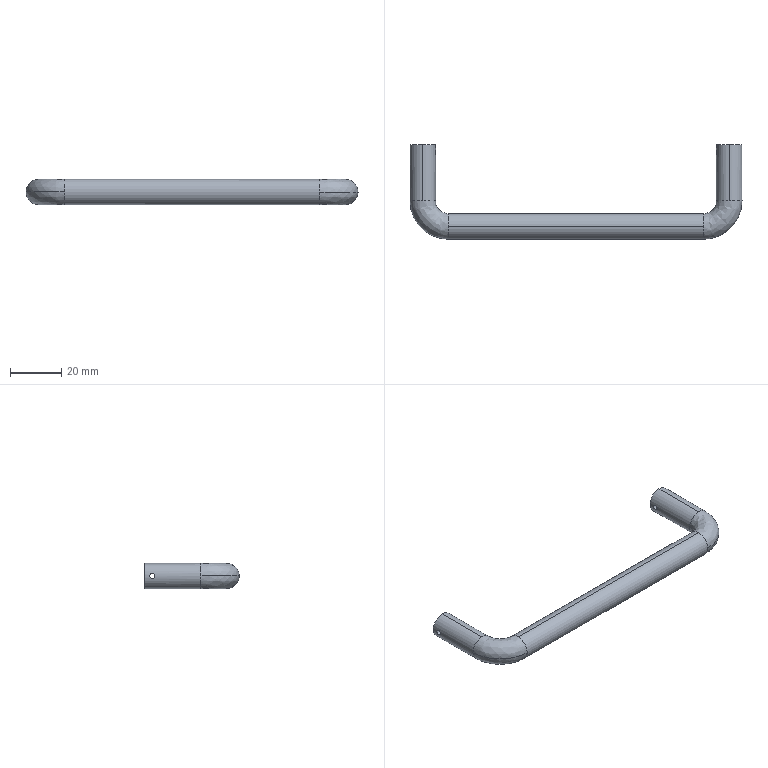Component | SolidWorks | ControlAssembly-1_UWAFN120-1_2_1-1 | 1 solid | 16 faces | box 130 x 37 x 10.01 mm | volume 13715 mm3 | cylinder 10 | spline 4 | plane 2 | commonest cylinder face diameters 10 x6 2 x4
STEP:
#1=COLOUR_RGB('',0.7922,0.8196,0.9333);
#2=FILL_AREA_STYLE_COLOUR('',#1);
#3=FILL_AREA_STYLE('',(#2));
#4=SURFACE_STYLE_FILL_AREA(#3);
#5=SURFACE_SIDE_STYLE('',(#4));
#6=SURFACE_STYLE_USAGE(.BOTH.,#5);
#7=PRESENTATION_STYLE_ASSIGNMENT((#6));
#8=CARTESIAN_POINT('',(19.707,0.8097,21.042));
#9=VERTEX_POINT('',#8);
#10=CARTESIAN_POINT('',(19.707,0.8097,21.121));
#11=VERTEX_POINT('',#10);
#12=CARTESIAN_POINT('',(19.707,0.8097,21.042));
#13=CARTESIAN_POINT('',(19.707,0.8149,21.042));
#14=CARTESIAN_POINT('',(19.707,0.82,21.043));
#15=CARTESIAN_POINT('',(19.706,0.8295,21.047));
#16=CARTESIAN_POINT('',(19.706,0.8339,21.05));
#17=CARTESIAN_POINT('',(19.705,0.8412,21.057));
#18=CARTESIAN_POINT('',(19.704,0.8441,21.061));
#19=CARTESIAN_POINT('',(19.703,0.848,21.071));
#20=CARTESIAN_POINT('',(19.703,0.8491,21.076));
#21=CARTESIAN_POINT('',(19.703,0.8491,21.086));
#22=CARTESIAN_POINT('',(19.703,0.848,21.092));
#23=CARTESIAN_POINT('',(19.704,0.8441,21.101));
#24=CARTESIAN_POINT('',(19.705,0.8411,21.105));
#25=CARTESIAN_POINT('',(19.706,0.8339,21.113));
#26=CARTESIAN_POINT('',(19.706,0.8295,21.116));
#27=CARTESIAN_POINT('',(19.707,0.82,21.12));
#28=CARTESIAN_POINT('',(19.707,0.8149,21.121));
#29=CARTESIAN_POINT('',(19.707,0.8097,21.121));
#30=B_SPLINE_CURVE_WITH_KNOTS('',3,(#12,#13,#14,#15,#16,#17,#18,#19,#20,#21,#22,#23,#24,#25,#26,#27,#28,#29),.UNSPECIFIED.,.F.,.F.,(4,2,2,2,2,2,2,2,4),(0.004702,0.005093,0.005485,0.005877,0.006269,0.00666,0.007052,0.007444,0.007836),.UNSPECIFIED.);
#31=EDGE_CURVE('',#9,#11,#30,.T.);
#32=ORIENTED_EDGE('',*,*,#31,.F.);
#33=CARTESIAN_POINT('',(20.093,0.8097,21.042));
#34=VERTEX_POINT('',#33);
#35=CARTESIAN_POINT('',(19.703,0.8097,21.042));
#36=DIRECTION('',(1.,0.,-0.00009864));
#37=VECTOR('',#36,39.37);
#38=LINE('',#35,#37);
#39=EDGE_CURVE('',#9,#34,#38,.T.);
#40=ORIENTED_EDGE('',*,*,#39,.T.);
#41=CARTESIAN_POINT('',(20.093,0.8097,21.121));
#42=VERTEX_POINT('',#41);
#43=CARTESIAN_POINT('',(20.093,0.8097,21.121));
#44=CARTESIAN_POINT('',(20.093,0.8149,21.121));
#45=CARTESIAN_POINT('',(20.093,0.82,21.119));
#46=CARTESIAN_POINT('',(20.094,0.8296,21.116));
#47=CARTESIAN_POINT('',(20.094,0.8339,21.113));
#48=CARTESIAN_POINT('',(20.095,0.8412,21.105));
#49=CARTESIAN_POINT('',(20.096,0.8441,21.101));
#50=CARTESIAN_POINT('',(20.097,0.848,21.091));
#51=CARTESIAN_POINT('',(20.097,0.8491,21.086));
#52=CARTESIAN_POINT('',(20.097,0.8491,21.076));
#53=CARTESIAN_POINT('',(20.097,0.848,21.071));
#54=CARTESIAN_POINT('',(20.096,0.8441,21.061));
#55=CARTESIAN_POINT('',(20.095,0.8412,21.057));
#56=CARTESIAN_POINT('',(20.094,0.8339,21.05));
#57=CARTESIAN_POINT('',(20.094,0.8295,21.047));
#58=CARTESIAN_POINT('',(20.093,0.82,21.043));
#59=CARTESIAN_POINT('',(20.093,0.8148,21.042));
#60=CARTESIAN_POINT('',(20.093,0.8097,21.042));
#61=B_SPLINE_CURVE_WITH_KNOTS('',3,(#43,#44,#45,#46,#47,#48,#49,#50,#51,#52,#53,#54,#55,#56,#57,#58,#59,#60),.UNSPECIFIED.,.F.,.F.,(4,2,2,2,2,2,2,2,4),(0.,0.0003918,0.0007836,0.001175,0.001567,0.001959,0.002351,0.002743,0.003134),.UNSPECIFIED.);
#62=EDGE_CURVE('',#42,#34,#61,.T.);
#63=ORIENTED_EDGE('',*,*,#62,.F.);
#64=CARTESIAN_POINT('',(19.703,0.8097,21.121));
#65=DIRECTION('',(1.,0.,-0.00009864));
#66=VECTOR('',#65,39.37);
#67=LINE('',#64,#66);
#68=EDGE_CURVE('',#11,#42,#67,.T.);
#69=ORIENTED_EDGE('',*,*,#68,.F.);
#70=EDGE_LOOP('',(#32,#40,#63,#69));
#71=FACE_OUTER_BOUND('',#70,.T.);
#72=CARTESIAN_POINT('',(19.703,0.8097,21.081));
#73=DIRECTION('',(1.,0.,-0.00009864));
#74=DIRECTION('',(0.00009864,0.,1.));
#75=AXIS2_PLACEMENT_3D('',#72,#73,#74);
#76=CYLINDRICAL_SURFACE('',#75,0.03937);
#77=ADVANCED_FACE('',(#71),#76,.F.);
#78=CARTESIAN_POINT('',(24.431,0.8097,21.041));
#79=VERTEX_POINT('',#78);
#80=CARTESIAN_POINT('',(24.431,0.8097,21.12));
#81=VERTEX_POINT('',#80);
#82=CARTESIAN_POINT('',(24.431,0.8097,21.041));
#83=CARTESIAN_POINT('',(24.431,0.8148,21.041));
#84=CARTESIAN_POINT('',(24.431,0.82,21.042));
#85=CARTESIAN_POINT('',(24.43,0.8295,21.046));
#86=CARTESIAN_POINT('',(24.43,0.8339,21.049));
#87=CARTESIAN_POINT('',(24.429,0.8412,21.056));
#88=CARTESIAN_POINT('',(24.428,0.8441,21.061));
#89=CARTESIAN_POINT('',(24.428,0.848,21.07));
#90=CARTESIAN_POINT('',(24.427,0.8491,21.075));
#91=CARTESIAN_POINT('',(24.427,0.8491,21.086));
#92=CARTESIAN_POINT('',(24.428,0.848,21.091));
#93=CARTESIAN_POINT('',(24.428,0.8441,21.101));
#94=CARTESIAN_POINT('',(24.429,0.8412,21.105));
#95=CARTESIAN_POINT('',(24.43,0.8339,21.112));
#96=CARTESIAN_POINT('',(24.43,0.8296,21.115));
#97=CARTESIAN_POINT('',(24.431,0.8201,21.119));
#98=CARTESIAN_POINT('',(24.431,0.8149,21.12));
#99=CARTESIAN_POINT('',(24.431,0.8097,21.12));
#100=B_SPLINE_CURVE_WITH_KNOTS('',3,(#82,#83,#84,#85,#86,#87,#88,#89,#90,#91,#92,#93,#94,#95,#96,#97,#98,#99),.UNSPECIFIED.,.F.,.F.,(4,2,2,2,2,2,2,2,4),(0.003134,0.003526,0.003918,0.004309,0.004701,0.005093,0.005485,0.005876,0.006268),.UNSPECIFIED.);
#101=EDGE_CURVE('',#79,#81,#100,.T.);
#102=ORIENTED_EDGE('',*,*,#101,.F.);
#103=CARTESIAN_POINT('',(24.817,0.8097,21.041));
#104=VERTEX_POINT('',#103);
#105=CARTESIAN_POINT('',(19.703,0.8097,21.042));
#106=DIRECTION('',(1.,0.,-0.00009864));
#107=VECTOR('',#106,39.37);
#108=LINE('',#105,#107);
#109=EDGE_CURVE('',#79,#104,#108,.T.);
#110=ORIENTED_EDGE('',*,*,#109,.T.);
#111=CARTESIAN_POINT('',(24.817,0.8097,21.12));
#112=VERTEX_POINT('',#111);
#113=CARTESIAN_POINT('',(24.817,0.8097,21.12));
#114=CARTESIAN_POINT('',(24.817,0.8149,21.12));
#115=CARTESIAN_POINT('',(24.817,0.82,21.119));
#116=CARTESIAN_POINT('',(24.818,0.8296,21.115));
#117=CARTESIAN_POINT('',(24.819,0.8339,21.112));
#118=CARTESIAN_POINT('',(24.82,0.8412,21.105));
#119=CARTESIAN_POINT('',(24.82,0.8441,21.101));
#120=CARTESIAN_POINT('',(24.821,0.848,21.091));
#121=CARTESIAN_POINT('',(24.821,0.8491,21.086));
#122=CARTESIAN_POINT('',(24.821,0.8491,21.076));
#123=CARTESIAN_POINT('',(24.821,0.848,21.07));
#124=CARTESIAN_POINT('',(24.82,0.8441,21.061));
#125=CARTESIAN_POINT('',(24.82,0.8412,21.056));
#126=CARTESIAN_POINT('',(24.819,0.8339,21.049));
#127=CARTESIAN_POINT('',(24.818,0.8295,21.046));
#128=CARTESIAN_POINT('',(24.817,0.82,21.042));
#129=CARTESIAN_POINT('',(24.817,0.8148,21.041));
#130=CARTESIAN_POINT('',(24.817,0.8097,21.041));
#131=B_SPLINE_CURVE_WITH_KNOTS('',3,(#113,#114,#115,#116,#117,#118,#119,#120,#121,#122,#123,#124,#125,#126,#127,#128,#129,#130),.UNSPECIFIED.,.F.,.F.,(4,2,2,2,2,2,2,2,4),(0.,0.0003918,0.0007836,0.001175,0.001567,0.001959,0.002351,0.002743,0.003134),.UNSPECIFIED.);
#132=EDGE_CURVE('',#112,#104,#131,.T.);
#133=ORIENTED_EDGE('',*,*,#132,.F.);
#134=CARTESIAN_POINT('',(19.703,0.8097,21.121));
#135=DIRECTION('',(1.,0.,-0.00009864));
#136=VECTOR('',#135,39.37);
#137=LINE('',#134,#136);
#138=EDGE_CURVE('',#81,#112,#137,.T.);
#139=ORIENTED_EDGE('',*,*,#138,.F.);
#140=EDGE_LOOP('',(#102,#110,#133,#139));
#141=FACE_OUTER_BOUND('',#140,.T.);
#142=CARTESIAN_POINT('',(19.703,0.8097,21.081));
#143=DIRECTION('',(1.,0.,-0.00009864));
#144=DIRECTION('',(0.00009864,0.,1.));
#145=AXIS2_PLACEMENT_3D('',#142,#143,#144);
#146=CYLINDRICAL_SURFACE('',#145,0.03937);
#147=ADVANCED_FACE('',(#141),#146,.F.);
#148=CARTESIAN_POINT('',(24.231,-0.5289,21.081));
#149=VERTEX_POINT('',#148);
#150=CARTESIAN_POINT('',(24.231,-0.332,21.278));
#151=VERTEX_POINT('',#150);
#152=CARTESIAN_POINT('',(24.231,-0.332,21.081));
#153=DIRECTION('',(-1.,-0.,0.00009864));
#154=DIRECTION('',(-0.00009864,-0.,-1.));
#155=AXIS2_PLACEMENT_3D('',#152,#153,#154);
#156=CIRCLE('',#155,0.1969);
#157=EDGE_CURVE('',#149,#151,#156,.T.);
#158=ORIENTED_EDGE('',*,*,#157,.T.);
#159=CARTESIAN_POINT('',(20.294,-0.332,21.278));
#160=VERTEX_POINT('',#159);
#161=CARTESIAN_POINT('',(22.262,-0.332,21.278));
#162=DIRECTION('',(-1.,-0.,0.00009864));
#163=VECTOR('',#162,39.37);
#164=LINE('',#161,#163);
#165=EDGE_CURVE('',#151,#160,#164,.T.);
#166=ORIENTED_EDGE('',*,*,#165,.T.);
#167=CARTESIAN_POINT('',(20.294,-0.5289,21.081));
#168=VERTEX_POINT('',#167);
#169=CARTESIAN_POINT('',(20.294,-0.332,21.081));
#170=DIRECTION('',(1.,0.,-0.00009864));
#171=DIRECTION('',(-0.00009864,-0.,-1.));
#172=AXIS2_PLACEMENT_3D('',#169,#170,#171);
#173=CIRCLE('',#172,0.1969);
#174=EDGE_CURVE('',#160,#168,#173,.T.);
#175=ORIENTED_EDGE('',*,*,#174,.T.);
#176=CARTESIAN_POINT('',(20.294,-0.332,20.884));
#177=VERTEX_POINT('',#176);
#178=CARTESIAN_POINT('',(20.294,-0.332,21.081));
#179=DIRECTION('',(1.,0.,-0.00009864));
#180=DIRECTION('',(-0.00009864,-0.,-1.));
#181=AXIS2_PLACEMENT_3D('',#178,#179,#180);
#182=CIRCLE('',#181,0.1969);
#183=EDGE_CURVE('',#168,#177,#182,.T.);
#184=ORIENTED_EDGE('',*,*,#183,.T.);
#185=CARTESIAN_POINT('',(24.231,-0.332,20.884));
#186=VERTEX_POINT('',#185);
#187=CARTESIAN_POINT('',(22.262,-0.332,20.884));
#188=DIRECTION('',(-1.,-0.,0.00009864));
#189=VECTOR('',#188,39.37);
#190=LINE('',#187,#189);
#191=EDGE_CURVE('',#186,#177,#190,.T.);
#192=ORIENTED_EDGE('',*,*,#191,.F.);
#193=CARTESIAN_POINT('',(24.231,-0.332,21.081));
#194=DIRECTION('',(-1.,-0.,0.00009864));
#195=DIRECTION('',(-0.00009864,-0.,-1.));
#196=AXIS2_PLACEMENT_3D('',#193,#194,#195);
#197=CIRCLE('',#196,0.1969);
#198=EDGE_CURVE('',#186,#149,#197,.T.);
#199=ORIENTED_EDGE('',*,*,#198,.T.);
#200=EDGE_LOOP('',(#158,#166,#175,#184,#192,#199));
#201=FACE_OUTER_BOUND('',#200,.T.);
#202=CARTESIAN_POINT('',(22.262,-0.332,21.081));
#203=DIRECTION('',(-1.,-0.,0.00009864));
#204=DIRECTION('',(-0.00009864,-0.,-1.));
#205=AXIS2_PLACEMENT_3D('',#202,#203,#204);
#206=CYLINDRICAL_SURFACE('',#205,0.1969);
#207=ADVANCED_FACE('',(#201),#206,.T.);
#208=CARTESIAN_POINT('',(24.231,-0.1352,21.081));
#209=VERTEX_POINT('',#208);
#210=CARTESIAN_POINT('',(24.231,-0.332,21.081));
#211=DIRECTION('',(-1.,-0.,0.00009864));
#212=DIRECTION('',(-0.00009864,-0.,-1.));
#213=AXIS2_PLACEMENT_3D('',#210,#211,#212);
#214=CIRCLE('',#213,0.1969);
#215=EDGE_CURVE('',#209,#186,#214,.T.);
#216=ORIENTED_EDGE('',*,*,#215,.F.);
#217=CARTESIAN_POINT('',(24.427,0.06167,21.081));
#218=VERTEX_POINT('',#217);
#219=CARTESIAN_POINT('',(24.231,0.06167,21.081));
#220=DIRECTION('',(0.00009864,0.,1.));
#221=DIRECTION('',(-1.,0.,0.00009864));
#222=AXIS2_PLACEMENT_3D('',#219,#220,#221);
#223=CIRCLE('',#222,0.1969);
#224=EDGE_CURVE('',#209,#218,#223,.T.);
#225=ORIENTED_EDGE('',*,*,#224,.T.);
#226=CARTESIAN_POINT('',(24.624,0.06167,20.884));
#227=VERTEX_POINT('',#226);
#228=CARTESIAN_POINT('',(24.624,0.06167,21.081));
#229=DIRECTION('',(-0.,-1.,0.));
#230=DIRECTION('',(1.,-0.,-0.00009864));
#231=AXIS2_PLACEMENT_3D('',#228,#229,#230);
#232=CIRCLE('',#231,0.1969);
#233=EDGE_CURVE('',#218,#227,#232,.T.);
#234=ORIENTED_EDGE('',*,*,#233,.T.);
#235=CARTESIAN_POINT('',(24.821,0.06167,21.081));
#236=VERTEX_POINT('',#235);
#237=CARTESIAN_POINT('',(24.624,0.06167,21.081));
#238=DIRECTION('',(-0.,-1.,0.));
#239=DIRECTION('',(1.,-0.,-0.00009864));
#240=AXIS2_PLACEMENT_3D('',#237,#238,#239);
#241=CIRCLE('',#240,0.1969);
#242=EDGE_CURVE('',#227,#236,#241,.T.);
#243=ORIENTED_EDGE('',*,*,#242,.T.);
#244=CARTESIAN_POINT('',(24.231,0.06167,21.081));
#245=DIRECTION('',(0.00009864,0.,1.));
#246=DIRECTION('',(-1.,-0.,0.00009864));
#247=AXIS2_PLACEMENT_3D('',#244,#245,#246);
#248=CIRCLE('',#247,0.5906);
#249=EDGE_CURVE('',#149,#236,#248,.T.);
#250=ORIENTED_EDGE('',*,*,#249,.F.);
#251=ORIENTED_EDGE('',*,*,#198,.F.);
#252=EDGE_LOOP('',(#216,#225,#234,#243,#250,#251));
#253=FACE_OUTER_BOUND('',#252,.T.);
#254=CARTESIAN_POINT('',(24.231,-0.5289,21.081));
#255=CARTESIAN_POINT('',(24.577,-0.5289,21.081));
#256=CARTESIAN_POINT('',(24.821,-0.2843,21.081));
#257=CARTESIAN_POINT('',(24.821,0.06167,21.081));
#258=CARTESIAN_POINT('',(24.231,-0.5289,20.687));
#259=CARTESIAN_POINT('',(24.577,-0.5289,20.687));
#260=CARTESIAN_POINT('',(24.821,-0.2843,20.687));
#261=CARTESIAN_POINT('',(24.821,0.06167,20.687));
#262=CARTESIAN_POINT('',(24.231,-0.1352,20.687));
#263=CARTESIAN_POINT('',(24.346,-0.1352,20.687));
#264=CARTESIAN_POINT('',(24.427,-0.05364,20.687));
#265=CARTESIAN_POINT('',(24.427,0.06167,20.687));
#266=CARTESIAN_POINT('',(24.231,-0.1352,21.081));
#267=CARTESIAN_POINT('',(24.346,-0.1352,21.081));
#268=CARTESIAN_POINT('',(24.427,-0.05364,21.081));
#269=CARTESIAN_POINT('',(24.427,0.06167,21.081));
#270=(BOUNDED_SURFACE()B_SPLINE_SURFACE(3,3,((#254,#255,#256,#257),(#258,#259,#260,#261),(#262,#263,#264,#265),(#266,#267,#268,#269)),.UNSPECIFIED.,.F.,.F.,.T.)B_SPLINE_SURFACE_WITH_KNOTS((4,4),(4,4),(0.,1.),(0.,1.),.UNSPECIFIED.)GEOMETRIC_REPRESENTATION_ITEM()RATIONAL_B_SPLINE_SURFACE(((1.,0.8047,0.8047,1.),(0.3333,0.2682,0.2682,0.3333),(0.3333,0.2682,0.2682,0.3333),(1.,0.8047,0.8047,1.)))REPRESENTATION_ITEM('')SURFACE());
#271=ADVANCED_FACE('',(#253),#270,.T.);
#272=CARTESIAN_POINT('',(20.294,-0.1352,21.081));
#273=VERTEX_POINT('',#272);
#274=CARTESIAN_POINT('',(20.294,-0.332,21.081));
#275=DIRECTION('',(1.,0.,-0.00009864));
#276=DIRECTION('',(-0.00009864,-0.,-1.));
#277=AXIS2_PLACEMENT_3D('',#274,#275,#276);
#278=CIRCLE('',#277,0.1969);
#279=EDGE_CURVE('',#273,#160,#278,.T.);
#280=ORIENTED_EDGE('',*,*,#279,.F.);
#281=CARTESIAN_POINT('',(20.097,0.06167,21.081));
#282=VERTEX_POINT('',#281);
#283=CARTESIAN_POINT('',(20.294,0.06167,21.081));
#284=DIRECTION('',(-0.00009864,-0.,-1.));
#285=DIRECTION('',(1.,0.,-0.00009864));
#286=AXIS2_PLACEMENT_3D('',#283,#284,#285);
#287=CIRCLE('',#286,0.1969);
#288=EDGE_CURVE('',#273,#282,#287,.T.);
#289=ORIENTED_EDGE('',*,*,#288,.T.);
#290=CARTESIAN_POINT('',(19.9,0.06167,21.278));
#291=VERTEX_POINT('',#290);
#292=CARTESIAN_POINT('',(19.9,0.06167,21.081));
#293=DIRECTION('',(0.,-1.,0.));
#294=DIRECTION('',(-1.,-0.,0.00009864));
#295=AXIS2_PLACEMENT_3D('',#292,#293,#294);
#296=CIRCLE('',#295,0.1969);
#297=EDGE_CURVE('',#282,#291,#296,.T.);
#298=ORIENTED_EDGE('',*,*,#297,.T.);
#299=CARTESIAN_POINT('',(19.703,0.06167,21.081));
#300=VERTEX_POINT('',#299);
#301=CARTESIAN_POINT('',(19.9,0.06167,21.081));
#302=DIRECTION('',(0.,-1.,0.));
#303=DIRECTION('',(-1.,-0.,0.00009864));
#304=AXIS2_PLACEMENT_3D('',#301,#302,#303);
#305=CIRCLE('',#304,0.1969);
#306=EDGE_CURVE('',#291,#300,#305,.T.);
#307=ORIENTED_EDGE('',*,*,#306,.T.);
#308=CARTESIAN_POINT('',(20.294,0.06167,21.081));
#309=DIRECTION('',(-0.00009864,-0.,-1.));
#310=DIRECTION('',(1.,0.,-0.00009864));
#311=AXIS2_PLACEMENT_3D('',#308,#309,#310);
#312=CIRCLE('',#311,0.5906);
#313=EDGE_CURVE('',#168,#300,#312,.T.);
#314=ORIENTED_EDGE('',*,*,#313,.F.);
#315=ORIENTED_EDGE('',*,*,#174,.F.);
#316=EDGE_LOOP('',(#280,#289,#298,#307,#314,#315));
#317=FACE_OUTER_BOUND('',#316,.T.);
#318=CARTESIAN_POINT('',(20.294,-0.5289,21.081));
#319=CARTESIAN_POINT('',(19.948,-0.5289,21.081));
#320=CARTESIAN_POINT('',(19.703,-0.2843,21.081));
#321=CARTESIAN_POINT('',(19.703,0.06167,21.081));
#322=CARTESIAN_POINT('',(20.294,-0.5289,21.475));
#323=CARTESIAN_POINT('',(19.948,-0.5289,21.475));
#324=CARTESIAN_POINT('',(19.703,-0.2843,21.475));
#325=CARTESIAN_POINT('',(19.703,0.06167,21.475));
#326=CARTESIAN_POINT('',(20.294,-0.1352,21.475));
#327=CARTESIAN_POINT('',(20.178,-0.1352,21.475));
#328=CARTESIAN_POINT('',(20.097,-0.05364,21.475));
#329=CARTESIAN_POINT('',(20.097,0.06167,21.475));
#330=CARTESIAN_POINT('',(20.294,-0.1352,21.081));
#331=CARTESIAN_POINT('',(20.178,-0.1352,21.081));
#332=CARTESIAN_POINT('',(20.097,-0.05364,21.081));
#333=CARTESIAN_POINT('',(20.097,0.06167,21.081));
#334=(BOUNDED_SURFACE()B_SPLINE_SURFACE(3,3,((#318,#319,#320,#321),(#322,#323,#324,#325),(#326,#327,#328,#329),(#330,#331,#332,#333)),.UNSPECIFIED.,.F.,.F.,.T.)B_SPLINE_SURFACE_WITH_KNOTS((4,4),(4,4),(0.,1.),(0.,1.),.UNSPECIFIED.)GEOMETRIC_REPRESENTATION_ITEM()RATIONAL_B_SPLINE_SURFACE(((1.,0.8047,0.8047,1.),(0.3333,0.2682,0.2682,0.3333),(0.3333,0.2682,0.2682,0.3333),(1.,0.8047,0.8047,1.)))REPRESENTATION_ITEM('')SURFACE());
#335=ADVANCED_FACE('',(#317),#334,.T.);
#336=CARTESIAN_POINT('',(24.431,0.8097,21.12));
#337=CARTESIAN_POINT('',(24.431,0.8045,21.12));
#338=CARTESIAN_POINT('',(24.431,0.7994,21.119));
#339=CARTESIAN_POINT('',(24.43,0.7898,21.115));
#340=CARTESIAN_POINT('',(24.43,0.7855,21.112));
#341=CARTESIAN_POINT('',(24.429,0.7782,21.105));
#342=CARTESIAN_POINT('',(24.428,0.7753,21.101));
#343=CARTESIAN_POINT('',(24.428,0.7714,21.091));
#344=CARTESIAN_POINT('',(24.427,0.7703,21.086));
#345=CARTESIAN_POINT('',(24.427,0.7703,21.076));
#346=CARTESIAN_POINT('',(24.428,0.7714,21.07));
#347=CARTESIAN_POINT('',(24.428,0.7753,21.061));
#348=CARTESIAN_POINT('',(24.429,0.7782,21.057));
#349=CARTESIAN_POINT('',(24.43,0.7855,21.049));
#350=CARTESIAN_POINT('',(24.43,0.7899,21.046));
#351=CARTESIAN_POINT('',(24.431,0.7994,21.042));
#352=CARTESIAN_POINT('',(24.431,0.8046,21.041));
#353=CARTESIAN_POINT('',(24.431,0.8097,21.041));
#354=B_SPLINE_CURVE_WITH_KNOTS('',3,(#336,#337,#338,#339,#340,#341,#342,#343,#344,#345,#346,#347,#348,#349,#350,#351,#352,#353),.UNSPECIFIED.,.F.,.F.,(4,2,2,2,2,2,2,2,4),(0.,0.0003918,0.0007836,0.001175,0.001567,0.001959,0.002351,0.002743,0.003134),.UNSPECIFIED.);
#355=EDGE_CURVE('',#81,#79,#354,.T.);
#356=ORIENTED_EDGE('',*,*,#355,.T.);
#357=ORIENTED_EDGE('',*,*,#101,.T.);
#358=EDGE_LOOP('',(#356,#357));
#359=FACE_BOUND('',#358,.T.);
#360=CARTESIAN_POINT('',(24.624,0.06167,21.278));
#361=VERTEX_POINT('',#360);
#362=CARTESIAN_POINT('',(24.624,0.06167,21.081));
#363=DIRECTION('',(-0.,-1.,0.));
#364=DIRECTION('',(1.,-0.,-0.00009864));
#365=AXIS2_PLACEMENT_3D('',#362,#363,#364);
#366=CIRCLE('',#365,0.1969);
#367=EDGE_CURVE('',#361,#218,#366,.T.);
#368=ORIENTED_EDGE('',*,*,#367,.F.);
#369=CARTESIAN_POINT('',(24.624,0.9278,21.278));
#370=VERTEX_POINT('',#369);
#371=CARTESIAN_POINT('',(24.624,0.9278,21.278));
#372=DIRECTION('',(-0.,1.,-0.));
#373=VECTOR('',#372,39.37);
#374=LINE('',#371,#373);
#375=EDGE_CURVE('',#361,#370,#374,.T.);
#376=ORIENTED_EDGE('',*,*,#375,.T.);
#377=CARTESIAN_POINT('',(24.624,0.9278,20.884));
#378=VERTEX_POINT('',#377);
#379=CARTESIAN_POINT('',(24.624,0.9278,21.081));
#380=DIRECTION('',(0.,-1.,0.));
#381=DIRECTION('',(-0.00009864,-0.,-1.));
#382=AXIS2_PLACEMENT_3D('',#379,#380,#381);
#383=CIRCLE('',#382,0.1969);
#384=EDGE_CURVE('',#370,#378,#383,.T.);
#385=ORIENTED_EDGE('',*,*,#384,.T.);
#386=CARTESIAN_POINT('',(24.624,0.9278,20.884));
#387=DIRECTION('',(-0.,1.,-0.));
#388=VECTOR('',#387,39.37);
#389=LINE('',#386,#388);
#390=EDGE_CURVE('',#227,#378,#389,.T.);
#391=ORIENTED_EDGE('',*,*,#390,.F.);
#392=ORIENTED_EDGE('',*,*,#233,.F.);
#393=EDGE_LOOP('',(#368,#376,#385,#391,#392));
#394=FACE_OUTER_BOUND('',#393,.T.);
#395=CARTESIAN_POINT('',(24.624,0.9278,21.081));
#396=DIRECTION('',(-0.,1.,-0.));
#397=DIRECTION('',(-0.00009864,-0.,-1.));
#398=AXIS2_PLACEMENT_3D('',#395,#396,#397);
#399=CYLINDRICAL_SURFACE('',#398,0.1969);
#400=ADVANCED_FACE('',(#359,#394),#399,.T.);
#401=CARTESIAN_POINT('',(19.707,0.8097,21.121));
#402=CARTESIAN_POINT('',(19.707,0.8046,21.121));
#403=CARTESIAN_POINT('',(19.707,0.7994,21.12));
#404=CARTESIAN_POINT('',(19.706,0.7898,21.116));
#405=CARTESIAN_POINT('',(19.706,0.7855,21.113));
#406=CARTESIAN_POINT('',(19.705,0.7782,21.105));
#407=CARTESIAN_POINT('',(19.704,0.7753,21.101));
#408=CARTESIAN_POINT('',(19.703,0.7714,21.091));
#409=CARTESIAN_POINT('',(19.703,0.7703,21.086));
#410=CARTESIAN_POINT('',(19.703,0.7703,21.076));
#411=CARTESIAN_POINT('',(19.703,0.7714,21.071));
#412=CARTESIAN_POINT('',(19.704,0.7753,21.061));
#413=CARTESIAN_POINT('',(19.705,0.7782,21.057));
#414=CARTESIAN_POINT('',(19.706,0.7855,21.05));
#415=CARTESIAN_POINT('',(19.706,0.7898,21.047));
#416=CARTESIAN_POINT('',(19.707,0.7994,21.043));
#417=CARTESIAN_POINT('',(19.707,0.8045,21.042));
#418=CARTESIAN_POINT('',(19.707,0.8097,21.042));
#419=B_SPLINE_CURVE_WITH_KNOTS('',3,(#401,#402,#403,#404,#405,#406,#407,#408,#409,#410,#411,#412,#413,#414,#415,#416,#417,#418),.UNSPECIFIED.,.F.,.F.,(4,2,2,2,2,2,2,2,4),(0.001568,0.001959,0.002351,0.002743,0.003135,0.003526,0.003918,0.00431,0.004702),.UNSPECIFIED.);
#420=EDGE_CURVE('',#11,#9,#419,.T.);
#421=ORIENTED_EDGE('',*,*,#420,.T.);
#422=ORIENTED_EDGE('',*,*,#31,.T.);
#423=EDGE_LOOP('',(#421,#422));
#424=FACE_BOUND('',#423,.T.);
#425=ORIENTED_EDGE('',*,*,#306,.F.);
#426=CARTESIAN_POINT('',(19.9,0.9278,21.278));
#427=VERTEX_POINT('',#426);
#428=CARTESIAN_POINT('',(19.9,0.9278,21.278));
#429=DIRECTION('',(-0.,1.,-0.));
#430=VECTOR('',#429,39.37);
#431=LINE('',#428,#430);
#432=EDGE_CURVE('',#291,#427,#431,.T.);
#433=ORIENTED_EDGE('',*,*,#432,.T.);
#434=CARTESIAN_POINT('',(19.9,0.9278,20.884));
#435=VERTEX_POINT('',#434);
#436=CARTESIAN_POINT('',(19.9,0.9278,21.081));
#437=DIRECTION('',(0.,-1.,0.));
#438=DIRECTION('',(-0.00009864,-0.,-1.));
#439=AXIS2_PLACEMENT_3D('',#436,#437,#438);
#440=CIRCLE('',#439,0.1969);
#441=EDGE_CURVE('',#427,#435,#440,.T.);
#442=ORIENTED_EDGE('',*,*,#441,.T.);
#443=CARTESIAN_POINT('',(19.9,0.06167,20.884));
#444=VERTEX_POINT('',#443);
#445=CARTESIAN_POINT('',(19.9,0.9278,20.884));
#446=DIRECTION('',(-0.,1.,-0.));
#447=VECTOR('',#446,39.37);
#448=LINE('',#445,#447);
#449=EDGE_CURVE('',#444,#435,#448,.T.);
#450=ORIENTED_EDGE('',*,*,#449,.F.);
#451=CARTESIAN_POINT('',(19.9,0.06167,21.081));
#452=DIRECTION('',(0.,-1.,0.));
#453=DIRECTION('',(-1.,-0.,0.00009864));
#454=AXIS2_PLACEMENT_3D('',#451,#452,#453);
#455=CIRCLE('',#454,0.1969);
#456=EDGE_CURVE('',#300,#444,#455,.T.);
#457=ORIENTED_EDGE('',*,*,#456,.F.);
#458=EDGE_LOOP('',(#425,#433,#442,#450,#457));
#459=FACE_OUTER_BOUND('',#458,.T.);
#460=CARTESIAN_POINT('',(19.9,0.9278,21.081));
#461=DIRECTION('',(-0.,1.,-0.));
#462=DIRECTION('',(-0.00009864,-0.,-1.));
#463=AXIS2_PLACEMENT_3D('',#460,#461,#462);
#464=CYLINDRICAL_SURFACE('',#463,0.1969);
#465=ADVANCED_FACE('',(#424,#459),#464,.T.);
#466=ORIENTED_EDGE('',*,*,#432,.F.);
#467=ORIENTED_EDGE('',*,*,#297,.F.);
#468=CARTESIAN_POINT('',(19.9,0.06167,21.081));
#469=DIRECTION('',(0.,-1.,0.));
#470=DIRECTION('',(-1.,-0.,0.00009864));
#471=AXIS2_PLACEMENT_3D('',#468,#469,#470);
#472=CIRCLE('',#471,0.1969);
#473=EDGE_CURVE('',#444,#282,#472,.T.);
#474=ORIENTED_EDGE('',*,*,#473,.F.);
#475=ORIENTED_EDGE('',*,*,#449,.T.);
#476=CARTESIAN_POINT('',(19.9,0.9278,21.081));
#477=DIRECTION('',(0.,-1.,0.));
#478=DIRECTION('',(-0.00009864,-0.,-1.));
#479=AXIS2_PLACEMENT_3D('',#476,#477,#478);
#480=CIRCLE('',#479,0.1969);
#481=EDGE_CURVE('',#435,#427,#480,.T.);
#482=ORIENTED_EDGE('',*,*,#481,.T.);
#483=EDGE_LOOP('',(#466,#467,#474,#475,#482));
#484=FACE_OUTER_BOUND('',#483,.T.);
#485=ORIENTED_EDGE('',*,*,#62,.T.);
#486=CARTESIAN_POINT('',(20.093,0.8097,21.042));
#487=CARTESIAN_POINT('',(20.093,0.8046,21.042));
#488=CARTESIAN_POINT('',(20.093,0.7994,21.043));
#489=CARTESIAN_POINT('',(20.094,0.7899,21.047));
#490=CARTESIAN_POINT('',(20.094,0.7855,21.05));
#491=CARTESIAN_POINT('',(20.095,0.7782,21.057));
#492=CARTESIAN_POINT('',(20.096,0.7753,21.061));
#493=CARTESIAN_POINT('',(20.097,0.7714,21.071));
#494=CARTESIAN_POINT('',(20.097,0.7703,21.076));
#495=CARTESIAN_POINT('',(20.097,0.7703,21.086));
#496=CARTESIAN_POINT('',(20.097,0.7714,21.091));
#497=CARTESIAN_POINT('',(20.096,0.7753,21.101));
#498=CARTESIAN_POINT('',(20.095,0.7782,21.105));
#499=CARTESIAN_POINT('',(20.094,0.7855,21.113));
#500=CARTESIAN_POINT('',(20.094,0.7898,21.116));
#501=CARTESIAN_POINT('',(20.093,0.7993,21.119));
#502=CARTESIAN_POINT('',(20.093,0.8045,21.121));
#503=CARTESIAN_POINT('',(20.093,0.8097,21.121));
#504=B_SPLINE_CURVE_WITH_KNOTS('',3,(#486,#487,#488,#489,#490,#491,#492,#493,#494,#495,#496,#497,#498,#499,#500,#501,#502,#503),.UNSPECIFIED.,.F.,.F.,(4,2,2,2,2,2,2,2,4),(0.003134,0.003526,0.003918,0.004309,0.004701,0.005093,0.005485,0.005876,0.006268),.UNSPECIFIED.);
#505=EDGE_CURVE('',#34,#42,#504,.T.);
#506=ORIENTED_EDGE('',*,*,#505,.T.);
#507=EDGE_LOOP('',(#485,#506));
#508=FACE_BOUND('',#507,.T.);
#509=CARTESIAN_POINT('',(19.9,0.9278,21.081));
#510=DIRECTION('',(-0.,1.,-0.));
#511=DIRECTION('',(-0.00009864,-0.,-1.));
#512=AXIS2_PLACEMENT_3D('',#509,#510,#511);
#513=CYLINDRICAL_SURFACE('',#512,0.1969);
#514=ADVANCED_FACE('',(#484,#508),#513,.T.);
#515=ORIENTED_EDGE('',*,*,#375,.F.);
#516=CARTESIAN_POINT('',(24.624,0.06167,21.081));
#517=DIRECTION('',(-0.,-1.,0.));
#518=DIRECTION('',(1.,-0.,-0.00009864));
#519=AXIS2_PLACEMENT_3D('',#516,#517,#518);
#520=CIRCLE('',#519,0.1969);
#521=EDGE_CURVE('',#236,#361,#520,.T.);
#522=ORIENTED_EDGE('',*,*,#521,.F.);
#523=ORIENTED_EDGE('',*,*,#242,.F.);
#524=ORIENTED_EDGE('',*,*,#390,.T.);
#525=CARTESIAN_POINT('',(24.624,0.9278,21.081));
#526=DIRECTION('',(0.,-1.,0.));
#527=DIRECTION('',(-0.00009864,-0.,-1.));
#528=AXIS2_PLACEMENT_3D('',#525,#526,#527);
#529=CIRCLE('',#528,0.1969);
#530=EDGE_CURVE('',#378,#370,#529,.T.);
#531=ORIENTED_EDGE('',*,*,#530,.T.);
#532=EDGE_LOOP('',(#515,#522,#523,#524,#531));
#533=FACE_OUTER_BOUND('',#532,.T.);
#534=ORIENTED_EDGE('',*,*,#132,.T.);
#535=CARTESIAN_POINT('',(24.817,0.8097,21.041));
#536=CARTESIAN_POINT('',(24.817,0.8046,21.041));
#537=CARTESIAN_POINT('',(24.817,0.7994,21.042));
#538=CARTESIAN_POINT('',(24.818,0.7899,21.046));
#539=CARTESIAN_POINT('',(24.819,0.7855,21.049));
#540=CARTESIAN_POINT('',(24.82,0.7782,21.056));
#541=CARTESIAN_POINT('',(24.82,0.7753,21.061));
#542=CARTESIAN_POINT('',(24.821,0.7714,21.07));
#543=CARTESIAN_POINT('',(24.821,0.7703,21.075));
#544=CARTESIAN_POINT('',(24.821,0.7703,21.086));
#545=CARTESIAN_POINT('',(24.821,0.7714,21.091));
#546=CARTESIAN_POINT('',(24.82,0.7753,21.101));
#547=CARTESIAN_POINT('',(24.82,0.7782,21.105));
#548=CARTESIAN_POINT('',(24.819,0.7855,21.112));
#549=CARTESIAN_POINT('',(24.818,0.7898,21.115));
#550=CARTESIAN_POINT('',(24.817,0.7993,21.119));
#551=CARTESIAN_POINT('',(24.817,0.8045,21.12));
#552=CARTESIAN_POINT('',(24.817,0.8097,21.12));
#553=B_SPLINE_CURVE_WITH_KNOTS('',3,(#535,#536,#537,#538,#539,#540,#541,#542,#543,#544,#545,#546,#547,#548,#549,#550,#551,#552),.UNSPECIFIED.,.F.,.F.,(4,2,2,2,2,2,2,2,4),(0.003134,0.003526,0.003918,0.004309,0.004701,0.005093,0.005485,0.005876,0.006268),.UNSPECIFIED.);
#554=EDGE_CURVE('',#104,#112,#553,.T.);
#555=ORIENTED_EDGE('',*,*,#554,.T.);
#556=EDGE_LOOP('',(#534,#555));
#557=FACE_BOUND('',#556,.T.);
#558=CARTESIAN_POINT('',(24.624,0.9278,21.081));
#559=DIRECTION('',(-0.,1.,-0.));
#560=DIRECTION('',(-0.00009864,-0.,-1.));
#561=AXIS2_PLACEMENT_3D('',#558,#559,#560);
#562=CYLINDRICAL_SURFACE('',#561,0.1969);
#563=ADVANCED_FACE('',(#533,#557),#562,.T.);
#564=ORIENTED_EDGE('',*,*,#165,.F.);
#565=CARTESIAN_POINT('',(24.231,-0.332,21.081));
#566=DIRECTION('',(-1.,-0.,0.00009864));
#567=DIRECTION('',(-0.00009864,-0.,-1.));
#568=AXIS2_PLACEMENT_3D('',#565,#566,#567);
#569=CIRCLE('',#568,0.1969);
#570=EDGE_CURVE('',#151,#209,#569,.T.);
#571=ORIENTED_EDGE('',*,*,#570,.T.);
#572=ORIENTED_EDGE('',*,*,#215,.T.);
#573=ORIENTED_EDGE('',*,*,#191,.T.);
#574=CARTESIAN_POINT('',(20.294,-0.332,21.081));
#575=DIRECTION('',(1.,0.,-0.00009864));
#576=DIRECTION('',(-0.00009864,-0.,-1.));
#577=AXIS2_PLACEMENT_3D('',#574,#575,#576);
#578=CIRCLE('',#577,0.1969);
#579=EDGE_CURVE('',#177,#273,#578,.T.);
#580=ORIENTED_EDGE('',*,*,#579,.T.);
#581=ORIENTED_EDGE('',*,*,#279,.T.);
#582=EDGE_LOOP('',(#564,#571,#572,#573,#580,#581));
#583=FACE_OUTER_BOUND('',#582,.T.);
#584=CARTESIAN_POINT('',(22.262,-0.332,21.081));
#585=DIRECTION('',(-1.,-0.,0.00009864));
#586=DIRECTION('',(-0.00009864,-0.,-1.));
#587=AXIS2_PLACEMENT_3D('',#584,#585,#586);
#588=CYLINDRICAL_SURFACE('',#587,0.1969);
#589=ADVANCED_FACE('',(#583),#588,.T.);
#590=ORIENTED_EDGE('',*,*,#224,.F.);
#591=ORIENTED_EDGE('',*,*,#570,.F.);
#592=ORIENTED_EDGE('',*,*,#157,.F.);
#593=ORIENTED_EDGE('',*,*,#249,.T.);
#594=ORIENTED_EDGE('',*,*,#521,.T.);
#595=ORIENTED_EDGE('',*,*,#367,.T.);
#596=EDGE_LOOP('',(#590,#591,#592,#593,#594,#595));
#597=FACE_OUTER_BOUND('',#596,.T.);
#598=CARTESIAN_POINT('',(24.231,-0.1352,21.081));
#599=CARTESIAN_POINT('',(24.346,-0.1352,21.081));
#600=CARTESIAN_POINT('',(24.427,-0.05364,21.081));
#601=CARTESIAN_POINT('',(24.427,0.06167,21.081));
#602=CARTESIAN_POINT('',(24.231,-0.1352,21.474));
#603=CARTESIAN_POINT('',(24.346,-0.1352,21.474));
#604=CARTESIAN_POINT('',(24.428,-0.05364,21.474));
#605=CARTESIAN_POINT('',(24.428,0.06167,21.474));
#606=CARTESIAN_POINT('',(24.231,-0.5289,21.474));
#607=CARTESIAN_POINT('',(24.577,-0.5289,21.474));
#608=CARTESIAN_POINT('',(24.821,-0.2843,21.474));
#609=CARTESIAN_POINT('',(24.821,0.06167,21.474));
#610=CARTESIAN_POINT('',(24.231,-0.5289,21.081));
#611=CARTESIAN_POINT('',(24.577,-0.5289,21.081));
#612=CARTESIAN_POINT('',(24.821,-0.2843,21.081));
#613=CARTESIAN_POINT('',(24.821,0.06167,21.081));
#614=(BOUNDED_SURFACE()B_SPLINE_SURFACE(3,3,((#598,#599,#600,#601),(#602,#603,#604,#605),(#606,#607,#608,#609),(#610,#611,#612,#613)),.UNSPECIFIED.,.F.,.F.,.T.)B_SPLINE_SURFACE_WITH_KNOTS((4,4),(4,4),(0.,1.),(0.,1.),.UNSPECIFIED.)GEOMETRIC_REPRESENTATION_ITEM()RATIONAL_B_SPLINE_SURFACE(((1.,0.8047,0.8047,1.),(0.3333,0.2682,0.2682,0.3333),(0.3333,0.2682,0.2682,0.3333),(1.,0.8047,0.8047,1.)))REPRESENTATION_ITEM('')SURFACE());
#615=ADVANCED_FACE('',(#597),#614,.T.);
#616=ORIENTED_EDGE('',*,*,#288,.F.);
#617=ORIENTED_EDGE('',*,*,#579,.F.);
#618=ORIENTED_EDGE('',*,*,#183,.F.);
#619=ORIENTED_EDGE('',*,*,#313,.T.);
#620=ORIENTED_EDGE('',*,*,#456,.T.);
#621=ORIENTED_EDGE('',*,*,#473,.T.);
#622=EDGE_LOOP('',(#616,#617,#618,#619,#620,#621));
#623=FACE_OUTER_BOUND('',#622,.T.);
#624=CARTESIAN_POINT('',(20.294,-0.1352,21.081));
#625=CARTESIAN_POINT('',(20.178,-0.1352,21.081));
#626=CARTESIAN_POINT('',(20.097,-0.05364,21.081));
#627=CARTESIAN_POINT('',(20.097,0.06167,21.081));
#628=CARTESIAN_POINT('',(20.294,-0.1352,20.687));
#629=CARTESIAN_POINT('',(20.178,-0.1352,20.687));
#630=CARTESIAN_POINT('',(20.097,-0.05364,20.687));
#631=CARTESIAN_POINT('',(20.097,0.06167,20.687));
#632=CARTESIAN_POINT('',(20.294,-0.5289,20.687));
#633=CARTESIAN_POINT('',(19.948,-0.5289,20.687));
#634=CARTESIAN_POINT('',(19.703,-0.2843,20.687));
#635=CARTESIAN_POINT('',(19.703,0.06167,20.687));
#636=CARTESIAN_POINT('',(20.294,-0.5289,21.081));
#637=CARTESIAN_POINT('',(19.948,-0.5289,21.081));
#638=CARTESIAN_POINT('',(19.703,-0.2843,21.081));
#639=CARTESIAN_POINT('',(19.703,0.06167,21.081));
#640=(BOUNDED_SURFACE()B_SPLINE_SURFACE(3,3,((#624,#625,#626,#627),(#628,#629,#630,#631),(#632,#633,#634,#635),(#636,#637,#638,#639)),.UNSPECIFIED.,.F.,.F.,.T.)B_SPLINE_SURFACE_WITH_KNOTS((4,4),(4,4),(0.,1.),(0.,1.),.UNSPECIFIED.)GEOMETRIC_REPRESENTATION_ITEM()RATIONAL_B_SPLINE_SURFACE(((1.,0.8047,0.8047,1.),(0.3333,0.2682,0.2682,0.3333),(0.3333,0.2682,0.2682,0.3333),(1.,0.8047,0.8047,1.)))REPRESENTATION_ITEM('')SURFACE());
#641=ADVANCED_FACE('',(#623),#640,.T.);
#642=ORIENTED_EDGE('',*,*,#530,.F.);
#643=ORIENTED_EDGE('',*,*,#384,.F.);
#644=EDGE_LOOP('',(#642,#643));
#645=FACE_OUTER_BOUND('',#644,.T.);
#646=CARTESIAN_POINT('',(24.624,0.9278,21.081));
#647=DIRECTION('',(0.,-1.,0.));
#648=DIRECTION('',(0.00009864,0.,1.));
#649=AXIS2_PLACEMENT_3D('',#646,#647,#648);
#650=PLANE('',#649);
#651=ADVANCED_FACE('',(#645),#650,.F.);
#652=ORIENTED_EDGE('',*,*,#481,.F.);
#653=ORIENTED_EDGE('',*,*,#441,.F.);
#654=EDGE_LOOP('',(#652,#653));
#655=FACE_OUTER_BOUND('',#654,.T.);
#656=CARTESIAN_POINT('',(24.624,0.9278,21.081));
#657=DIRECTION('',(0.,-1.,0.));
#658=DIRECTION('',(0.00009864,0.,1.));
#659=AXIS2_PLACEMENT_3D('',#656,#657,#658);
#660=PLANE('',#659);
#661=ADVANCED_FACE('',(#655),#660,.F.);
#662=ORIENTED_EDGE('',*,*,#109,.F.);
#663=ORIENTED_EDGE('',*,*,#355,.F.);
#664=ORIENTED_EDGE('',*,*,#138,.T.);
#665=ORIENTED_EDGE('',*,*,#554,.F.);
#666=EDGE_LOOP('',(#662,#663,#664,#665));
#667=FACE_OUTER_BOUND('',#666,.T.);
#668=CARTESIAN_POINT('',(19.703,0.8097,21.081));
#669=DIRECTION('',(1.,0.,-0.00009864));
#670=DIRECTION('',(0.00009864,0.,1.));
#671=AXIS2_PLACEMENT_3D('',#668,#669,#670);
#672=CYLINDRICAL_SURFACE('',#671,0.03937);
#673=ADVANCED_FACE('',(#667),#672,.F.);
#674=ORIENTED_EDGE('',*,*,#39,.F.);
#675=ORIENTED_EDGE('',*,*,#420,.F.);
#676=ORIENTED_EDGE('',*,*,#68,.T.);
#677=ORIENTED_EDGE('',*,*,#505,.F.);
#678=EDGE_LOOP('',(#674,#675,#676,#677));
#679=FACE_OUTER_BOUND('',#678,.T.);
#680=CARTESIAN_POINT('',(19.703,0.8097,21.081));
#681=DIRECTION('',(1.,0.,-0.00009864));
#682=DIRECTION('',(0.00009864,0.,1.));
#683=AXIS2_PLACEMENT_3D('',#680,#681,#682);
#684=CYLINDRICAL_SURFACE('',#683,0.03937);
#685=ADVANCED_FACE('',(#679),#684,.F.);
#686=CLOSED_SHELL('',(#77,#147,#207,#271,#335,#400,#465,#514,#563,#589,#615,#641,#651,#661,#673,#685));
#687=MANIFOLD_SOLID_BREP('',#686);
#688=STYLED_ITEM('',(#7),#687);
#689=(LENGTH_UNIT()NAMED_UNIT(*)SI_UNIT($,.METRE.));
#690=LENGTH_MEASURE_WITH_UNIT(LENGTH_MEASURE(0.0254),#689);
#691=DIMENSIONAL_EXPONENTS(1.,0.,0.,0.,0.,0.,0.);
#692=(CONVERSION_BASED_UNIT('',#690)LENGTH_UNIT()NAMED_UNIT(#691));
#693=UNCERTAINTY_MEASURE_WITH_UNIT(LENGTH_MEASURE(0.00001),#692,'','');
#694=(NAMED_UNIT(*)PLANE_ANGLE_UNIT()SI_UNIT($,.RADIAN.));
#695=(NAMED_UNIT(*)SI_UNIT($,.STERADIAN.)SOLID_ANGLE_UNIT());
#696=(GEOMETRIC_REPRESENTATION_CONTEXT(3)GLOBAL_UNCERTAINTY_ASSIGNED_CONTEXT((#693))GLOBAL_UNIT_ASSIGNED_CONTEXT((#692,#694,#695))REPRESENTATION_CONTEXT('',''));
#697=MECHANICAL_DESIGN_GEOMETRIC_PRESENTATION_REPRESENTATION('',(#688),#696);
#698=CARTESIAN_POINT('',(0.,0.,0.));
#699=DIRECTION('',(0.,0.,1.));
#700=DIRECTION('',(1.,0.,0.));
#701=AXIS2_PLACEMENT_3D('',#698,#699,#700);
#702=(LENGTH_UNIT()NAMED_UNIT(*)SI_UNIT($,.METRE.));
#703=LENGTH_MEASURE_WITH_UNIT(LENGTH_MEASURE(0.0254),#702);
#704=DIMENSIONAL_EXPONENTS(1.,0.,0.,0.,0.,0.,0.);
#705=(CONVERSION_BASED_UNIT('',#703)LENGTH_UNIT()NAMED_UNIT(#704));
#706=UNCERTAINTY_MEASURE_WITH_UNIT(LENGTH_MEASURE(0.00001),#705,'','');
#707=(NAMED_UNIT(*)PLANE_ANGLE_UNIT()SI_UNIT($,.RADIAN.));
#708=(NAMED_UNIT(*)SI_UNIT($,.STERADIAN.)SOLID_ANGLE_UNIT());
#709=(GEOMETRIC_REPRESENTATION_CONTEXT(3)GLOBAL_UNCERTAINTY_ASSIGNED_CONTEXT((#706))GLOBAL_UNIT_ASSIGNED_CONTEXT((#705,#707,#708))REPRESENTATION_CONTEXT('',''));
#710=ADVANCED_BREP_SHAPE_REPRESENTATION('',(#687,#701),#709);
#711=PRESENTATION_LAYER_ASSIGNMENT('','',(#688));